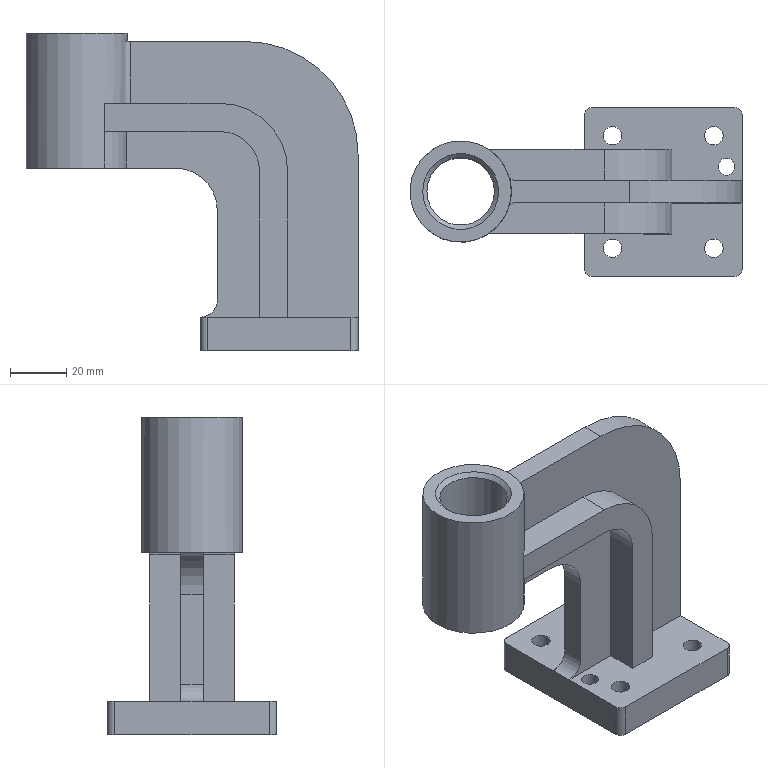Component | NX | BRACKET | 1 solid | 48 faces | volume 139454 mm3 | plane 25 | cylinder 22 | cone 1 | commonest cylinder face diameters 5 x4 6.6 x4 36 x2 48 x2 28 x2 6 x2 4 x2 30 x1